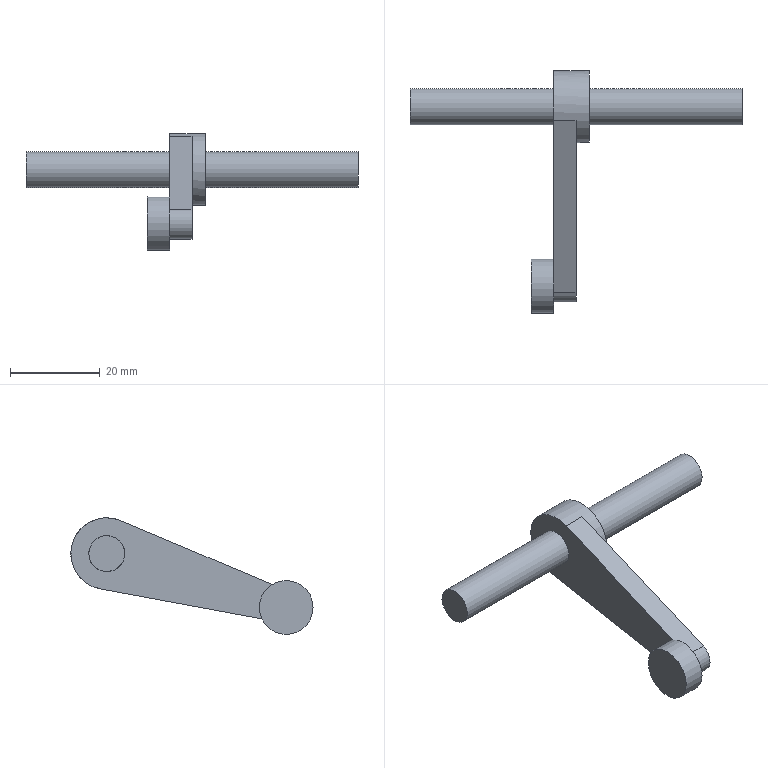Component | NX | DRIVEN_ROLLER | 3 solids | 17 faces | box 74 x 54 x 26 mm | volume 7500 mm3 | plane 10 | cylinder 7 | commonest cylinder face diameters 3 x2 8 x2 12 x1 7 x1 16 x1
STEP:
#1=CARTESIAN_POINT('',(0.,0.,0.));
#2=DIRECTION('',(0.,0.,1.));
#3=DIRECTION('',(1.,0.,0.));
#4=AXIS2_PLACEMENT_3D('',#1,#2,#3);
#5=CARTESIAN_POINT('',(25.,6.,197.818));
#6=VERTEX_POINT('',#5);
#7=CARTESIAN_POINT('',(25.,0.,197.818));
#8=DIRECTION('',(1.,0.,0.));
#9=DIRECTION('',(0.,1.,0.));
#10=AXIS2_PLACEMENT_3D('',#7,#8,#9);
#11=CIRCLE('',#10,6.);
#12=CARTESIAN_POINT('',(25.,0.,197.818));
#13=DIRECTION('',(-1.,0.,0.));
#14=DIRECTION('',(0.,0.,1.));
#15=AXIS2_PLACEMENT_3D('',#12,#13,#14);
#16=CYLINDRICAL_SURFACE('',#15,6.);
#17=CARTESIAN_POINT('',(7.854,0.));
#18=DIRECTION('',(-1.,0.));
#19=VECTOR('',#18,1.);
#20=LINE('',#17,#19);
#21=(GEOMETRIC_REPRESENTATION_CONTEXT(2)PARAMETRIC_REPRESENTATION_CONTEXT()REPRESENTATION_CONTEXT('',''));
#22=DEFINITIONAL_REPRESENTATION('',(#20),#21);
#23=PCURVE('',#16,#22);
#24=CARTESIAN_POINT('',(25.,0.,197.818));
#25=DIRECTION('',(1.,0.,0.));
#26=DIRECTION('',(0.,0.,-1.));
#27=AXIS2_PLACEMENT_3D('',#24,#25,#26);
#28=PLANE('',#27);
#29=CARTESIAN_POINT('',(0.,0.));
#30=DIRECTION('',(0.,1.));
#31=AXIS2_PLACEMENT_2D('',#29,#30);
#32=CIRCLE('',#31,6.);
#33=(GEOMETRIC_REPRESENTATION_CONTEXT(2)PARAMETRIC_REPRESENTATION_CONTEXT()REPRESENTATION_CONTEXT('',''));
#34=DEFINITIONAL_REPRESENTATION('',(#32),#33);
#35=PCURVE('',#28,#34);
#36=SURFACE_CURVE('',#11,(#23,#35),.PCURVE_S1.);
#37=EDGE_CURVE('',#6,#6,#36,.T.);
#38=ORIENTED_EDGE('',*,*,#37,.F.);
#39=CARTESIAN_POINT('',(20.,6.,197.818));
#40=VERTEX_POINT('',#39);
#41=CARTESIAN_POINT('',(25.,6.,197.818));
#42=CARTESIAN_POINT('',(20.,6.,197.818));
#43=B_SPLINE_CURVE_WITH_KNOTS('',1,(#41,#42),.UNSPECIFIED.,.F.,.F.,(2,2),(0.,5.),.PIECEWISE_BEZIER_KNOTS.);
#44=CARTESIAN_POINT('',(7.854,0.));
#45=DIRECTION('',(0.,1.));
#46=VECTOR('',#45,1.);
#47=LINE('',#44,#46);
#48=(GEOMETRIC_REPRESENTATION_CONTEXT(2)PARAMETRIC_REPRESENTATION_CONTEXT()REPRESENTATION_CONTEXT('',''));
#49=DEFINITIONAL_REPRESENTATION('',(#47),#48);
#50=PCURVE('',#16,#49);
#51=CARTESIAN_POINT('',(1.571,0.));
#52=DIRECTION('',(0.,1.));
#53=VECTOR('',#52,1.);
#54=LINE('',#51,#53);
#55=(GEOMETRIC_REPRESENTATION_CONTEXT(2)PARAMETRIC_REPRESENTATION_CONTEXT()REPRESENTATION_CONTEXT('',''));
#56=DEFINITIONAL_REPRESENTATION('',(#54),#55);
#57=PCURVE('',#16,#56);
#58=SEAM_CURVE('',#43,(#50,#57),.PCURVE_S1.);
#59=EDGE_CURVE('',#6,#40,#58,.T.);
#60=ORIENTED_EDGE('',*,*,#59,.T.);
#61=CARTESIAN_POINT('',(20.,0.,197.818));
#62=DIRECTION('',(1.,0.,0.));
#63=DIRECTION('',(0.,1.,0.));
#64=AXIS2_PLACEMENT_3D('',#61,#62,#63);
#65=CIRCLE('',#64,6.);
#66=CARTESIAN_POINT('',(7.854,5.));
#67=DIRECTION('',(-1.,0.));
#68=VECTOR('',#67,1.);
#69=LINE('',#66,#68);
#70=(GEOMETRIC_REPRESENTATION_CONTEXT(2)PARAMETRIC_REPRESENTATION_CONTEXT()REPRESENTATION_CONTEXT('',''));
#71=DEFINITIONAL_REPRESENTATION('',(#69),#70);
#72=PCURVE('',#16,#71);
#73=CARTESIAN_POINT('',(20.,0.,197.818));
#74=DIRECTION('',(1.,0.,0.));
#75=DIRECTION('',(0.,0.,-1.));
#76=AXIS2_PLACEMENT_3D('',#73,#74,#75);
#77=PLANE('',#76);
#78=CARTESIAN_POINT('',(0.,0.));
#79=DIRECTION('',(0.,1.));
#80=AXIS2_PLACEMENT_2D('',#78,#79);
#81=CIRCLE('',#80,6.);
#82=(GEOMETRIC_REPRESENTATION_CONTEXT(2)PARAMETRIC_REPRESENTATION_CONTEXT()REPRESENTATION_CONTEXT('',''));
#83=DEFINITIONAL_REPRESENTATION('',(#81),#82);
#84=PCURVE('',#77,#83);
#85=SURFACE_CURVE('',#65,(#72,#84),.PCURVE_S1.);
#86=EDGE_CURVE('',#40,#40,#85,.T.);
#87=ORIENTED_EDGE('',*,*,#86,.T.);
#88=ORIENTED_EDGE('',*,*,#59,.F.);
#89=EDGE_LOOP('',(#38,#60,#87,#88));
#90=FACE_BOUND('',#89,.T.);
#91=ADVANCED_FACE('',(#90),#16,.T.);
#92=CARTESIAN_POINT('',(25.,1.5,197.818));
#93=VERTEX_POINT('',#92);
#94=CARTESIAN_POINT('',(25.,0.,197.818));
#95=DIRECTION('',(1.,0.,0.));
#96=DIRECTION('',(0.,1.,0.));
#97=AXIS2_PLACEMENT_3D('',#94,#95,#96);
#98=CIRCLE('',#97,1.5);
#99=CARTESIAN_POINT('',(0.,0.));
#100=DIRECTION('',(0.,1.));
#101=AXIS2_PLACEMENT_2D('',#99,#100);
#102=CIRCLE('',#101,1.5);
#103=(GEOMETRIC_REPRESENTATION_CONTEXT(2)PARAMETRIC_REPRESENTATION_CONTEXT()REPRESENTATION_CONTEXT('',''));
#104=DEFINITIONAL_REPRESENTATION('',(#102),#103);
#105=PCURVE('',#28,#104);
#106=CARTESIAN_POINT('',(30.,0.,197.818));
#107=DIRECTION('',(-1.,0.,0.));
#108=DIRECTION('',(0.,0.,1.));
#109=AXIS2_PLACEMENT_3D('',#106,#107,#108);
#110=CYLINDRICAL_SURFACE('',#109,1.5);
#111=CARTESIAN_POINT('',(7.854,5.));
#112=DIRECTION('',(-1.,0.));
#113=VECTOR('',#112,1.);
#114=LINE('',#111,#113);
#115=(GEOMETRIC_REPRESENTATION_CONTEXT(2)PARAMETRIC_REPRESENTATION_CONTEXT()REPRESENTATION_CONTEXT('',''));
#116=DEFINITIONAL_REPRESENTATION('',(#114),#115);
#117=PCURVE('',#110,#116);
#118=SURFACE_CURVE('',#98,(#105,#117),.PCURVE_S1.);
#119=EDGE_CURVE('',#93,#93,#118,.T.);
#120=ORIENTED_EDGE('',*,*,#119,.F.);
#121=EDGE_LOOP('',(#120));
#122=FACE_BOUND('',#121,.T.);
#123=ORIENTED_EDGE('',*,*,#37,.T.);
#124=EDGE_LOOP('',(#123));
#125=FACE_BOUND('',#124,.T.);
#126=ADVANCED_FACE('',(#122,#125),#28,.T.);
#127=ORIENTED_EDGE('',*,*,#86,.F.);
#128=EDGE_LOOP('',(#127));
#129=FACE_BOUND('',#128,.T.);
#130=ADVANCED_FACE('',(#129),#77,.F.);
#131=CARTESIAN_POINT('',(30.,1.5,197.818));
#132=VERTEX_POINT('',#131);
#133=CARTESIAN_POINT('',(30.,0.,197.818));
#134=DIRECTION('',(1.,0.,0.));
#135=DIRECTION('',(0.,1.,0.));
#136=AXIS2_PLACEMENT_3D('',#133,#134,#135);
#137=CIRCLE('',#136,1.5);
#138=CARTESIAN_POINT('',(7.854,0.));
#139=DIRECTION('',(-1.,0.));
#140=VECTOR('',#139,1.);
#141=LINE('',#138,#140);
#142=(GEOMETRIC_REPRESENTATION_CONTEXT(2)PARAMETRIC_REPRESENTATION_CONTEXT()REPRESENTATION_CONTEXT('',''));
#143=DEFINITIONAL_REPRESENTATION('',(#141),#142);
#144=PCURVE('',#110,#143);
#145=CARTESIAN_POINT('',(30.,0.,197.818));
#146=DIRECTION('',(1.,0.,0.));
#147=DIRECTION('',(0.,0.,-1.));
#148=AXIS2_PLACEMENT_3D('',#145,#146,#147);
#149=PLANE('',#148);
#150=CARTESIAN_POINT('',(0.,0.));
#151=DIRECTION('',(0.,1.));
#152=AXIS2_PLACEMENT_2D('',#150,#151);
#153=CIRCLE('',#152,1.5);
#154=(GEOMETRIC_REPRESENTATION_CONTEXT(2)PARAMETRIC_REPRESENTATION_CONTEXT()REPRESENTATION_CONTEXT('',''));
#155=DEFINITIONAL_REPRESENTATION('',(#153),#154);
#156=PCURVE('',#149,#155);
#157=SURFACE_CURVE('',#137,(#144,#156),.PCURVE_S1.);
#158=EDGE_CURVE('',#132,#132,#157,.T.);
#159=ORIENTED_EDGE('',*,*,#158,.F.);
#160=CARTESIAN_POINT('',(30.,1.5,197.818));
#161=CARTESIAN_POINT('',(25.,1.5,197.818));
#162=B_SPLINE_CURVE_WITH_KNOTS('',1,(#160,#161),.UNSPECIFIED.,.F.,.F.,(2,2),(0.,5.),.PIECEWISE_BEZIER_KNOTS.);
#163=CARTESIAN_POINT('',(7.854,0.));
#164=DIRECTION('',(0.,1.));
#165=VECTOR('',#164,1.);
#166=LINE('',#163,#165);
#167=(GEOMETRIC_REPRESENTATION_CONTEXT(2)PARAMETRIC_REPRESENTATION_CONTEXT()REPRESENTATION_CONTEXT('',''));
#168=DEFINITIONAL_REPRESENTATION('',(#166),#167);
#169=PCURVE('',#110,#168);
#170=CARTESIAN_POINT('',(1.571,0.));
#171=DIRECTION('',(0.,1.));
#172=VECTOR('',#171,1.);
#173=LINE('',#170,#172);
#174=(GEOMETRIC_REPRESENTATION_CONTEXT(2)PARAMETRIC_REPRESENTATION_CONTEXT()REPRESENTATION_CONTEXT('',''));
#175=DEFINITIONAL_REPRESENTATION('',(#173),#174);
#176=PCURVE('',#110,#175);
#177=SEAM_CURVE('',#162,(#169,#176),.PCURVE_S1.);
#178=EDGE_CURVE('',#132,#93,#177,.T.);
#179=ORIENTED_EDGE('',*,*,#178,.T.);
#180=ORIENTED_EDGE('',*,*,#119,.T.);
#181=ORIENTED_EDGE('',*,*,#178,.F.);
#182=EDGE_LOOP('',(#159,#179,#180,#181));
#183=FACE_BOUND('',#182,.T.);
#184=ADVANCED_FACE('',(#183),#110,.T.);
#185=ORIENTED_EDGE('',*,*,#158,.T.);
#186=EDGE_LOOP('',(#185));
#187=FACE_BOUND('',#186,.T.);
#188=ADVANCED_FACE('',(#187),#149,.T.);
#189=CLOSED_SHELL('',(#91,#126,#130,#184,#188));
#190=MANIFOLD_SOLID_BREP('',#189);
#191=(LENGTH_UNIT()NAMED_UNIT(*)SI_UNIT(.MILLI.,.METRE.));
#192=UNCERTAINTY_MEASURE_WITH_UNIT(LENGTH_MEASURE(0.00001),#191,'','');
#193=(NAMED_UNIT(*)PLANE_ANGLE_UNIT()SI_UNIT($,.RADIAN.));
#194=(NAMED_UNIT(*)SI_UNIT($,.STERADIAN.)SOLID_ANGLE_UNIT());
#195=(GEOMETRIC_REPRESENTATION_CONTEXT(3)GLOBAL_UNCERTAINTY_ASSIGNED_CONTEXT((#192))GLOBAL_UNIT_ASSIGNED_CONTEXT((#191,#193,#194))REPRESENTATION_CONTEXT('',''));
#196=ADVANCED_BREP_SHAPE_REPRESENTATION('',(#4,#190),#195);
#197=CARTESIAN_POINT('',(0.,0.,0.));
#198=DIRECTION('',(0.,0.,1.));
#199=DIRECTION('',(1.,0.,0.));
#200=AXIS2_PLACEMENT_3D('',#197,#198,#199);
#201=CARTESIAN_POINT('',(0.,0.,0.));
#202=DIRECTION('',(0.,0.,1.));
#203=DIRECTION('',(1.,0.,0.));
#204=AXIS2_PLACEMENT_3D('',#201,#202,#203);
#205=CARTESIAN_POINT('',(0.,0.,0.));
#206=DIRECTION('',(0.,0.,1.));
#207=DIRECTION('',(1.,0.,0.));
#208=AXIS2_PLACEMENT_3D('',#205,#206,#207);
#209=(LENGTH_UNIT()NAMED_UNIT(*)SI_UNIT(.MILLI.,.METRE.));
#210=UNCERTAINTY_MEASURE_WITH_UNIT(LENGTH_MEASURE(0.000005),#209,'','');
#211=(NAMED_UNIT(*)PLANE_ANGLE_UNIT()SI_UNIT($,.RADIAN.));
#212=(NAMED_UNIT(*)SI_UNIT($,.STERADIAN.)SOLID_ANGLE_UNIT());
#213=(GEOMETRIC_REPRESENTATION_CONTEXT(3)GLOBAL_UNCERTAINTY_ASSIGNED_CONTEXT((#210))GLOBAL_UNIT_ASSIGNED_CONTEXT((#209,#211,#212))REPRESENTATION_CONTEXT('',''));
#214=SHAPE_REPRESENTATION('',(#4,#200,#204,#208),#213);
#215=ITEM_DEFINED_TRANSFORMATION('','',#4,#200);
#216=(REPRESENTATION_RELATIONSHIP('','',#196,#214)REPRESENTATION_RELATIONSHIP_WITH_TRANSFORMATION(#215)SHAPE_REPRESENTATION_RELATIONSHIP());
#217=CARTESIAN_POINT('',(25.,-1.361,201.043));
#218=VERTEX_POINT('',#217);
#219=CARTESIAN_POINT('',(25.,0.6386,194.377));
#220=VERTEX_POINT('',#219);
#221=CARTESIAN_POINT('',(25.,0.,197.818));
#222=DIRECTION('',(1.,0.,0.));
#223=DIRECTION('',(0.,1.,0.));
#224=AXIS2_PLACEMENT_3D('',#221,#222,#223);
#225=CIRCLE('',#224,3.5);
#226=CARTESIAN_POINT('',(30.,0.,197.818));
#227=DIRECTION('',(-1.,0.,0.));
#228=DIRECTION('',(0.,0.,1.));
#229=AXIS2_PLACEMENT_3D('',#226,#227,#228);
#230=CYLINDRICAL_SURFACE('',#229,3.5);
#231=CARTESIAN_POINT('',(7.854,5.));
#232=DIRECTION('',(-1.,0.));
#233=VECTOR('',#232,1.);
#234=LINE('',#231,#233);
#235=(GEOMETRIC_REPRESENTATION_CONTEXT(2)PARAMETRIC_REPRESENTATION_CONTEXT()REPRESENTATION_CONTEXT('',''));
#236=DEFINITIONAL_REPRESENTATION('',(#234),#235);
#237=PCURVE('',#230,#236);
#238=CARTESIAN_POINT('',(25.,0.,197.818));
#239=DIRECTION('',(1.,0.,0.));
#240=DIRECTION('',(0.,0.,-1.));
#241=AXIS2_PLACEMENT_3D('',#238,#239,#240);
#242=PLANE('',#241);
#243=CARTESIAN_POINT('',(0.,0.));
#244=DIRECTION('',(0.,1.));
#245=AXIS2_PLACEMENT_2D('',#243,#244);
#246=CIRCLE('',#245,3.5);
#247=(GEOMETRIC_REPRESENTATION_CONTEXT(2)PARAMETRIC_REPRESENTATION_CONTEXT()REPRESENTATION_CONTEXT('',''));
#248=DEFINITIONAL_REPRESENTATION('',(#246),#247);
#249=PCURVE('',#242,#248);
#250=SURFACE_CURVE('',#225,(#237,#249),.PCURVE_S1.);
#251=EDGE_CURVE('',#218,#220,#250,.T.);
#252=ORIENTED_EDGE('',*,*,#251,.T.);
#253=CARTESIAN_POINT('',(30.,0.6386,194.377));
#254=VERTEX_POINT('',#253);
#255=CARTESIAN_POINT('',(30.,0.6386,194.377));
#256=DIRECTION('',(-1.,0.,0.));
#257=VECTOR('',#256,1.);
#258=LINE('',#255,#257);
#259=CARTESIAN_POINT('',(2.958,0.));
#260=DIRECTION('',(0.,1.));
#261=VECTOR('',#260,1.);
#262=LINE('',#259,#261);
#263=(GEOMETRIC_REPRESENTATION_CONTEXT(2)PARAMETRIC_REPRESENTATION_CONTEXT()REPRESENTATION_CONTEXT('',''));
#264=DEFINITIONAL_REPRESENTATION('',(#262),#263);
#265=PCURVE('',#230,#264);
#266=CARTESIAN_POINT('',(30.,0.6386,194.377));
#267=DIRECTION('',(0.,-0.1825,0.9832));
#268=DIRECTION('',(0.,-0.9832,-0.1825));
#269=AXIS2_PLACEMENT_3D('',#266,#267,#268);
#270=PLANE('',#269);
#271=CARTESIAN_POINT('',(0.,0.));
#272=DIRECTION('',(0.,-1.));
#273=VECTOR('',#272,1.);
#274=LINE('',#271,#273);
#275=(GEOMETRIC_REPRESENTATION_CONTEXT(2)PARAMETRIC_REPRESENTATION_CONTEXT()REPRESENTATION_CONTEXT('',''));
#276=DEFINITIONAL_REPRESENTATION('',(#274),#275);
#277=PCURVE('',#270,#276);
#278=SURFACE_CURVE('',#258,(#265,#277),.PCURVE_S1.);
#279=EDGE_CURVE('',#254,#220,#278,.T.);
#280=ORIENTED_EDGE('',*,*,#279,.F.);
#281=CARTESIAN_POINT('',(30.,-1.361,201.043));
#282=VERTEX_POINT('',#281);
#283=CARTESIAN_POINT('',(30.,0.,197.818));
#284=DIRECTION('',(1.,0.,0.));
#285=DIRECTION('',(0.,1.,0.));
#286=AXIS2_PLACEMENT_3D('',#283,#284,#285);
#287=CIRCLE('',#286,3.5);
#288=CARTESIAN_POINT('',(7.854,0.));
#289=DIRECTION('',(-1.,0.));
#290=VECTOR('',#289,1.);
#291=LINE('',#288,#290);
#292=(GEOMETRIC_REPRESENTATION_CONTEXT(2)PARAMETRIC_REPRESENTATION_CONTEXT()REPRESENTATION_CONTEXT('',''));
#293=DEFINITIONAL_REPRESENTATION('',(#291),#292);
#294=PCURVE('',#230,#293);
#295=CARTESIAN_POINT('',(30.,0.,197.818));
#296=DIRECTION('',(1.,0.,0.));
#297=DIRECTION('',(0.,0.,-1.));
#298=AXIS2_PLACEMENT_3D('',#295,#296,#297);
#299=PLANE('',#298);
#300=CARTESIAN_POINT('',(0.,0.));
#301=DIRECTION('',(0.,1.));
#302=AXIS2_PLACEMENT_2D('',#300,#301);
#303=CIRCLE('',#302,3.5);
#304=(GEOMETRIC_REPRESENTATION_CONTEXT(2)PARAMETRIC_REPRESENTATION_CONTEXT()REPRESENTATION_CONTEXT('',''));
#305=DEFINITIONAL_REPRESENTATION('',(#303),#304);
#306=PCURVE('',#299,#305);
#307=SURFACE_CURVE('',#287,(#294,#306),.PCURVE_S1.);
#308=EDGE_CURVE('',#282,#254,#307,.T.);
#309=ORIENTED_EDGE('',*,*,#308,.F.);
#310=CARTESIAN_POINT('',(30.,-1.361,201.043));
#311=DIRECTION('',(-1.,0.,0.));
#312=VECTOR('',#311,1.);
#313=LINE('',#310,#312);
#314=CARTESIAN_POINT('',(5.884,0.));
#315=DIRECTION('',(0.,1.));
#316=VECTOR('',#315,1.);
#317=LINE('',#314,#316);
#318=(GEOMETRIC_REPRESENTATION_CONTEXT(2)PARAMETRIC_REPRESENTATION_CONTEXT()REPRESENTATION_CONTEXT('',''));
#319=DEFINITIONAL_REPRESENTATION('',(#317),#318);
#320=PCURVE('',#230,#319);
#321=CARTESIAN_POINT('',(30.,36.889,217.189));
#322=DIRECTION('',(0.,0.3889,-0.9213));
#323=DIRECTION('',(0.,0.9213,0.3889));
#324=AXIS2_PLACEMENT_3D('',#321,#322,#323);
#325=PLANE('',#324);
#326=CARTESIAN_POINT('',(-41.518,0.));
#327=DIRECTION('',(0.,-1.));
#328=VECTOR('',#327,1.);
#329=LINE('',#326,#328);
#330=(GEOMETRIC_REPRESENTATION_CONTEXT(2)PARAMETRIC_REPRESENTATION_CONTEXT()REPRESENTATION_CONTEXT('',''));
#331=DEFINITIONAL_REPRESENTATION('',(#329),#330);
#332=PCURVE('',#325,#331);
#333=SURFACE_CURVE('',#313,(#320,#332),.PCURVE_S1.);
#334=EDGE_CURVE('',#282,#218,#333,.T.);
#335=ORIENTED_EDGE('',*,*,#334,.T.);
#336=EDGE_LOOP('',(#252,#280,#309,#335));
#337=FACE_BOUND('',#336,.T.);
#338=ADVANCED_FACE('',(#337),#230,.T.);
#339=CARTESIAN_POINT('',(25.,41.46,201.953));
#340=VERTEX_POINT('',#339);
#341=CARTESIAN_POINT('',(25.,0.6386,194.377));
#342=DIRECTION('',(0.,0.9832,0.1825));
#343=VECTOR('',#342,1.);
#344=LINE('',#341,#343);
#345=CARTESIAN_POINT('',(0.,-5.));
#346=DIRECTION('',(-1.,0.));
#347=VECTOR('',#346,1.);
#348=LINE('',#345,#347);
#349=(GEOMETRIC_REPRESENTATION_CONTEXT(2)PARAMETRIC_REPRESENTATION_CONTEXT()REPRESENTATION_CONTEXT('',''));
#350=DEFINITIONAL_REPRESENTATION('',(#348),#349);
#351=PCURVE('',#270,#350);
#352=CARTESIAN_POINT('',(3.441,0.6386));
#353=DIRECTION('',(-0.1825,0.9832));
#354=VECTOR('',#353,1.);
#355=LINE('',#352,#354);
#356=(GEOMETRIC_REPRESENTATION_CONTEXT(2)PARAMETRIC_REPRESENTATION_CONTEXT()REPRESENTATION_CONTEXT('',''));
#357=DEFINITIONAL_REPRESENTATION('',(#355),#356);
#358=PCURVE('',#242,#357);
#359=SURFACE_CURVE('',#344,(#351,#358),.PCURVE_S1.);
#360=EDGE_CURVE('',#220,#340,#359,.T.);
#361=ORIENTED_EDGE('',*,*,#360,.T.);
#362=CARTESIAN_POINT('',(30.,41.46,201.953));
#363=VERTEX_POINT('',#362);
#364=CARTESIAN_POINT('',(30.,41.46,201.953));
#365=DIRECTION('',(-1.,0.,0.));
#366=VECTOR('',#365,1.);
#367=LINE('',#364,#366);
#368=CARTESIAN_POINT('',(-41.518,0.));
#369=DIRECTION('',(0.,-1.));
#370=VECTOR('',#369,1.);
#371=LINE('',#368,#370);
#372=(GEOMETRIC_REPRESENTATION_CONTEXT(2)PARAMETRIC_REPRESENTATION_CONTEXT()REPRESENTATION_CONTEXT('',''));
#373=DEFINITIONAL_REPRESENTATION('',(#371),#372);
#374=PCURVE('',#270,#373);
#375=CARTESIAN_POINT('',(30.,40.,209.818));
#376=DIRECTION('',(-1.,0.,0.));
#377=DIRECTION('',(0.,0.,1.));
#378=AXIS2_PLACEMENT_3D('',#375,#376,#377);
#379=CYLINDRICAL_SURFACE('',#378,8.);
#380=CARTESIAN_POINT('',(9.241,0.));
#381=DIRECTION('',(0.,1.));
#382=VECTOR('',#381,1.);
#383=LINE('',#380,#382);
#384=(GEOMETRIC_REPRESENTATION_CONTEXT(2)PARAMETRIC_REPRESENTATION_CONTEXT()REPRESENTATION_CONTEXT('',''));
#385=DEFINITIONAL_REPRESENTATION('',(#383),#384);
#386=PCURVE('',#379,#385);
#387=SURFACE_CURVE('',#367,(#374,#386),.PCURVE_S1.);
#388=EDGE_CURVE('',#363,#340,#387,.T.);
#389=ORIENTED_EDGE('',*,*,#388,.F.);
#390=CARTESIAN_POINT('',(30.,0.6386,194.377));
#391=DIRECTION('',(0.,0.9832,0.1825));
#392=VECTOR('',#391,1.);
#393=LINE('',#390,#392);
#394=CARTESIAN_POINT('',(0.,0.));
#395=DIRECTION('',(-1.,0.));
#396=VECTOR('',#395,1.);
#397=LINE('',#394,#396);
#398=(GEOMETRIC_REPRESENTATION_CONTEXT(2)PARAMETRIC_REPRESENTATION_CONTEXT()REPRESENTATION_CONTEXT('',''));
#399=DEFINITIONAL_REPRESENTATION('',(#397),#398);
#400=PCURVE('',#270,#399);
#401=CARTESIAN_POINT('',(3.441,0.6386));
#402=DIRECTION('',(-0.1825,0.9832));
#403=VECTOR('',#402,1.);
#404=LINE('',#401,#403);
#405=(GEOMETRIC_REPRESENTATION_CONTEXT(2)PARAMETRIC_REPRESENTATION_CONTEXT()REPRESENTATION_CONTEXT('',''));
#406=DEFINITIONAL_REPRESENTATION('',(#404),#405);
#407=PCURVE('',#299,#406);
#408=SURFACE_CURVE('',#393,(#400,#407),.PCURVE_S1.);
#409=EDGE_CURVE('',#254,#363,#408,.T.);
#410=ORIENTED_EDGE('',*,*,#409,.F.);
#411=ORIENTED_EDGE('',*,*,#279,.T.);
#412=EDGE_LOOP('',(#361,#389,#410,#411));
#413=FACE_BOUND('',#412,.T.);
#414=ADVANCED_FACE('',(#413),#270,.F.);
#415=CARTESIAN_POINT('',(25.,36.889,217.189));
#416=VERTEX_POINT('',#415);
#417=CARTESIAN_POINT('',(25.,40.,209.818));
#418=DIRECTION('',(1.,0.,0.));
#419=DIRECTION('',(0.,1.,0.));
#420=AXIS2_PLACEMENT_3D('',#417,#418,#419);
#421=CIRCLE('',#420,8.);
#422=CARTESIAN_POINT('',(14.137,5.));
#423=DIRECTION('',(-1.,0.));
#424=VECTOR('',#423,1.);
#425=LINE('',#422,#424);
#426=(GEOMETRIC_REPRESENTATION_CONTEXT(2)PARAMETRIC_REPRESENTATION_CONTEXT()REPRESENTATION_CONTEXT('',''));
#427=DEFINITIONAL_REPRESENTATION('',(#425),#426);
#428=PCURVE('',#379,#427);
#429=CARTESIAN_POINT('',(-12.,40.));
#430=DIRECTION('',(0.,1.));
#431=AXIS2_PLACEMENT_2D('',#429,#430);
#432=CIRCLE('',#431,8.);
#433=(GEOMETRIC_REPRESENTATION_CONTEXT(2)PARAMETRIC_REPRESENTATION_CONTEXT()REPRESENTATION_CONTEXT('',''));
#434=DEFINITIONAL_REPRESENTATION('',(#432),#433);
#435=PCURVE('',#242,#434);
#436=SURFACE_CURVE('',#421,(#428,#435),.PCURVE_S1.);
#437=EDGE_CURVE('',#340,#416,#436,.T.);
#438=ORIENTED_EDGE('',*,*,#437,.T.);
#439=CARTESIAN_POINT('',(30.,36.889,217.189));
#440=VERTEX_POINT('',#439);
#441=CARTESIAN_POINT('',(30.,36.889,217.189));
#442=DIRECTION('',(-1.,0.,0.));
#443=VECTOR('',#442,1.);
#444=LINE('',#441,#443);
#445=CARTESIAN_POINT('',(5.884,0.));
#446=DIRECTION('',(0.,1.));
#447=VECTOR('',#446,1.);
#448=LINE('',#445,#447);
#449=(GEOMETRIC_REPRESENTATION_CONTEXT(2)PARAMETRIC_REPRESENTATION_CONTEXT()REPRESENTATION_CONTEXT('',''));
#450=DEFINITIONAL_REPRESENTATION('',(#448),#449);
#451=PCURVE('',#379,#450);
#452=CARTESIAN_POINT('',(-0.,0.));
#453=DIRECTION('',(0.,-1.));
#454=VECTOR('',#453,1.);
#455=LINE('',#452,#454);
#456=(GEOMETRIC_REPRESENTATION_CONTEXT(2)PARAMETRIC_REPRESENTATION_CONTEXT()REPRESENTATION_CONTEXT('',''));
#457=DEFINITIONAL_REPRESENTATION('',(#455),#456);
#458=PCURVE('',#325,#457);
#459=SURFACE_CURVE('',#444,(#451,#458),.PCURVE_S1.);
#460=EDGE_CURVE('',#440,#416,#459,.T.);
#461=ORIENTED_EDGE('',*,*,#460,.F.);
#462=CARTESIAN_POINT('',(33.,36.889,217.189));
#463=VERTEX_POINT('',#462);
#464=CARTESIAN_POINT('',(33.,36.889,217.189));
#465=CARTESIAN_POINT('',(30.,36.889,217.189));
#466=B_SPLINE_CURVE_WITH_KNOTS('',1,(#464,#465),.UNSPECIFIED.,.F.,.F.,(2,2),(-3.,0.),.PIECEWISE_BEZIER_KNOTS.);
#467=CARTESIAN_POINT('',(5.884,0.));
#468=DIRECTION('',(0.,1.));
#469=VECTOR('',#468,1.);
#470=LINE('',#467,#469);
#471=(GEOMETRIC_REPRESENTATION_CONTEXT(2)PARAMETRIC_REPRESENTATION_CONTEXT()REPRESENTATION_CONTEXT('',''));
#472=DEFINITIONAL_REPRESENTATION('',(#470),#471);
#473=PCURVE('',#379,#472);
#474=CARTESIAN_POINT('',(12.167,0.));
#475=DIRECTION('',(0.,1.));
#476=VECTOR('',#475,1.);
#477=LINE('',#474,#476);
#478=(GEOMETRIC_REPRESENTATION_CONTEXT(2)PARAMETRIC_REPRESENTATION_CONTEXT()REPRESENTATION_CONTEXT('',''));
#479=DEFINITIONAL_REPRESENTATION('',(#477),#478);
#480=PCURVE('',#379,#479);
#481=SEAM_CURVE('',#466,(#473,#480),.PCURVE_S1.);
#482=EDGE_CURVE('',#463,#440,#481,.T.);
#483=ORIENTED_EDGE('',*,*,#482,.F.);
#484=CARTESIAN_POINT('',(33.,47.866,211.278));
#485=VERTEX_POINT('',#484);
#486=CARTESIAN_POINT('',(33.,40.,209.818));
#487=DIRECTION('',(1.,0.,0.));
#488=DIRECTION('',(0.,0.9832,0.1825));
#489=AXIS2_PLACEMENT_3D('',#486,#487,#488);
#490=CIRCLE('',#489,8.);
#491=CARTESIAN_POINT('',(7.67,-3.));
#492=DIRECTION('',(-1.,0.));
#493=VECTOR('',#492,1.);
#494=LINE('',#491,#493);
#495=(GEOMETRIC_REPRESENTATION_CONTEXT(2)PARAMETRIC_REPRESENTATION_CONTEXT()REPRESENTATION_CONTEXT('',''));
#496=DEFINITIONAL_REPRESENTATION('',(#494),#495);
#497=PCURVE('',#379,#496);
#498=CARTESIAN_POINT('',(33.,40.,209.818));
#499=DIRECTION('',(1.,0.,0.));
#500=DIRECTION('',(0.,0.,-1.));
#501=AXIS2_PLACEMENT_3D('',#498,#499,#500);
#502=PLANE('',#501);
#503=CARTESIAN_POINT('',(0.,0.));
#504=DIRECTION('',(-0.1825,0.9832));
#505=AXIS2_PLACEMENT_2D('',#503,#504);
#506=CIRCLE('',#505,8.);
#507=(GEOMETRIC_REPRESENTATION_CONTEXT(2)PARAMETRIC_REPRESENTATION_CONTEXT()REPRESENTATION_CONTEXT('',''));
#508=DEFINITIONAL_REPRESENTATION('',(#506),#507);
#509=PCURVE('',#502,#508);
#510=SURFACE_CURVE('',#490,(#497,#509),.PCURVE_S1.);
#511=EDGE_CURVE('',#485,#463,#510,.T.);
#512=ORIENTED_EDGE('',*,*,#511,.F.);
#513=CARTESIAN_POINT('',(33.,40.,209.818));
#514=DIRECTION('',(1.,0.,0.));
#515=DIRECTION('',(0.,0.9832,0.1825));
#516=AXIS2_PLACEMENT_3D('',#513,#514,#515);
#517=CIRCLE('',#516,8.);
#518=CARTESIAN_POINT('',(13.954,-3.));
#519=DIRECTION('',(-1.,0.));
#520=VECTOR('',#519,1.);
#521=LINE('',#518,#520);
#522=(GEOMETRIC_REPRESENTATION_CONTEXT(2)PARAMETRIC_REPRESENTATION_CONTEXT()REPRESENTATION_CONTEXT('',''));
#523=DEFINITIONAL_REPRESENTATION('',(#521),#522);
#524=PCURVE('',#379,#523);
#525=CARTESIAN_POINT('',(0.,0.));
#526=DIRECTION('',(-0.1825,0.9832));
#527=AXIS2_PLACEMENT_2D('',#525,#526);
#528=CIRCLE('',#527,8.);
#529=(GEOMETRIC_REPRESENTATION_CONTEXT(2)PARAMETRIC_REPRESENTATION_CONTEXT()REPRESENTATION_CONTEXT('',''));
#530=DEFINITIONAL_REPRESENTATION('',(#528),#529);
#531=PCURVE('',#502,#530);
#532=SURFACE_CURVE('',#517,(#524,#531),.PCURVE_S1.);
#533=EDGE_CURVE('',#463,#485,#532,.T.);
#534=ORIENTED_EDGE('',*,*,#533,.F.);
#535=ORIENTED_EDGE('',*,*,#482,.T.);
#536=CARTESIAN_POINT('',(30.,40.,209.818));
#537=DIRECTION('',(-1.,0.,0.));
#538=DIRECTION('',(0.,0.9832,0.1825));
#539=AXIS2_PLACEMENT_3D('',#536,#537,#538);
#540=CIRCLE('',#539,8.);
#541=CARTESIAN_POINT('',(7.67,0.));
#542=DIRECTION('',(1.,0.));
#543=VECTOR('',#542,1.);
#544=LINE('',#541,#543);
#545=(GEOMETRIC_REPRESENTATION_CONTEXT(2)PARAMETRIC_REPRESENTATION_CONTEXT()REPRESENTATION_CONTEXT('',''));
#546=DEFINITIONAL_REPRESENTATION('',(#544),#545);
#547=PCURVE('',#379,#546);
#548=CARTESIAN_POINT('',(-13.46,47.866));
#549=CARTESIAN_POINT('',(0.1641,50.394));
#550=CARTESIAN_POINT('',(-4.458,37.331));
#551=CARTESIAN_POINT('',(-9.081,24.269));
#552=CARTESIAN_POINT('',(-18.082,34.803));
#553=CARTESIAN_POINT('',(-27.084,45.337));
#554=CARTESIAN_POINT('',(-13.46,47.866));
#555=(BOUNDED_CURVE()B_SPLINE_CURVE(2,(#548,#549,#550,#551,#552,#553,#554),.UNSPECIFIED.,.T.,.F.)B_SPLINE_CURVE_WITH_KNOTS((1,2,2,2,2,1),(-2.094,0.,2.094,4.189,6.283,8.378),.UNSPECIFIED.)CURVE()GEOMETRIC_REPRESENTATION_ITEM()RATIONAL_B_SPLINE_CURVE((1.,0.5,1.,0.5,1.,0.5,1.))REPRESENTATION_ITEM(''));
#556=(GEOMETRIC_REPRESENTATION_CONTEXT(2)PARAMETRIC_REPRESENTATION_CONTEXT()REPRESENTATION_CONTEXT('',''));
#557=DEFINITIONAL_REPRESENTATION('',(#555),#556);
#558=PCURVE('',#299,#557);
#559=SURFACE_CURVE('',#540,(#547,#558),.PCURVE_S1.);
#560=EDGE_CURVE('',#363,#440,#559,.T.);
#561=ORIENTED_EDGE('',*,*,#560,.F.);
#562=ORIENTED_EDGE('',*,*,#388,.T.);
#563=EDGE_LOOP('',(#438,#461,#483,#512,#534,#535,#561,#562));
#564=FACE_BOUND('',#563,.T.);
#565=ADVANCED_FACE('',(#564),#379,.T.);
#566=CARTESIAN_POINT('',(30.,1.5,197.818));
#567=VERTEX_POINT('',#566);
#568=CARTESIAN_POINT('',(30.,0.,197.818));
#569=DIRECTION('',(1.,0.,0.));
#570=DIRECTION('',(0.,1.,0.));
#571=AXIS2_PLACEMENT_3D('',#568,#569,#570);
#572=CIRCLE('',#571,1.5);
#573=CARTESIAN_POINT('',(30.,0.,197.818));
#574=DIRECTION('',(-1.,0.,0.));
#575=DIRECTION('',(0.,0.,1.));
#576=AXIS2_PLACEMENT_3D('',#573,#574,#575);
#577=CYLINDRICAL_SURFACE('',#576,1.5);
#578=CARTESIAN_POINT('',(7.854,0.));
#579=DIRECTION('',(-1.,0.));
#580=VECTOR('',#579,1.);
#581=LINE('',#578,#580);
#582=(GEOMETRIC_REPRESENTATION_CONTEXT(2)PARAMETRIC_REPRESENTATION_CONTEXT()REPRESENTATION_CONTEXT('',''));
#583=DEFINITIONAL_REPRESENTATION('',(#581),#582);
#584=PCURVE('',#577,#583);
#585=CARTESIAN_POINT('',(0.,0.));
#586=DIRECTION('',(0.,1.));
#587=AXIS2_PLACEMENT_2D('',#585,#586);
#588=CIRCLE('',#587,1.5);
#589=(GEOMETRIC_REPRESENTATION_CONTEXT(2)PARAMETRIC_REPRESENTATION_CONTEXT()REPRESENTATION_CONTEXT('',''));
#590=DEFINITIONAL_REPRESENTATION('',(#588),#589);
#591=PCURVE('',#299,#590);
#592=SURFACE_CURVE('',#572,(#584,#591),.PCURVE_S1.);
#593=EDGE_CURVE('',#567,#567,#592,.T.);
#594=ORIENTED_EDGE('',*,*,#593,.F.);
#595=CARTESIAN_POINT('',(25.,1.5,197.818));
#596=VERTEX_POINT('',#595);
#597=CARTESIAN_POINT('',(30.,1.5,197.818));
#598=CARTESIAN_POINT('',(25.,1.5,197.818));
#599=B_SPLINE_CURVE_WITH_KNOTS('',1,(#597,#598),.UNSPECIFIED.,.F.,.F.,(2,2),(0.,5.),.PIECEWISE_BEZIER_KNOTS.);
#600=CARTESIAN_POINT('',(7.854,0.));
#601=DIRECTION('',(0.,1.));
#602=VECTOR('',#601,1.);
#603=LINE('',#600,#602);
#604=(GEOMETRIC_REPRESENTATION_CONTEXT(2)PARAMETRIC_REPRESENTATION_CONTEXT()REPRESENTATION_CONTEXT('',''));
#605=DEFINITIONAL_REPRESENTATION('',(#603),#604);
#606=PCURVE('',#577,#605);
#607=CARTESIAN_POINT('',(1.571,0.));
#608=DIRECTION('',(0.,1.));
#609=VECTOR('',#608,1.);
#610=LINE('',#607,#609);
#611=(GEOMETRIC_REPRESENTATION_CONTEXT(2)PARAMETRIC_REPRESENTATION_CONTEXT()REPRESENTATION_CONTEXT('',''));
#612=DEFINITIONAL_REPRESENTATION('',(#610),#611);
#613=PCURVE('',#577,#612);
#614=SEAM_CURVE('',#599,(#606,#613),.PCURVE_S1.);
#615=EDGE_CURVE('',#567,#596,#614,.T.);
#616=ORIENTED_EDGE('',*,*,#615,.T.);
#617=CARTESIAN_POINT('',(25.,0.,197.818));
#618=DIRECTION('',(1.,0.,0.));
#619=DIRECTION('',(0.,1.,0.));
#620=AXIS2_PLACEMENT_3D('',#617,#618,#619);
#621=CIRCLE('',#620,1.5);
#622=CARTESIAN_POINT('',(7.854,5.));
#623=DIRECTION('',(-1.,0.));
#624=VECTOR('',#623,1.);
#625=LINE('',#622,#624);
#626=(GEOMETRIC_REPRESENTATION_CONTEXT(2)PARAMETRIC_REPRESENTATION_CONTEXT()REPRESENTATION_CONTEXT('',''));
#627=DEFINITIONAL_REPRESENTATION('',(#625),#626);
#628=PCURVE('',#577,#627);
#629=CARTESIAN_POINT('',(0.,0.));
#630=DIRECTION('',(0.,1.));
#631=AXIS2_PLACEMENT_2D('',#629,#630);
#632=CIRCLE('',#631,1.5);
#633=(GEOMETRIC_REPRESENTATION_CONTEXT(2)PARAMETRIC_REPRESENTATION_CONTEXT()REPRESENTATION_CONTEXT('',''));
#634=DEFINITIONAL_REPRESENTATION('',(#632),#633);
#635=PCURVE('',#242,#634);
#636=SURFACE_CURVE('',#621,(#628,#635),.PCURVE_S1.);
#637=EDGE_CURVE('',#596,#596,#636,.T.);
#638=ORIENTED_EDGE('',*,*,#637,.T.);
#639=ORIENTED_EDGE('',*,*,#615,.F.);
#640=EDGE_LOOP('',(#594,#616,#638,#639));
#641=FACE_BOUND('',#640,.F.);
#642=ADVANCED_FACE('',(#641),#577,.F.);
#643=CARTESIAN_POINT('',(25.,36.889,217.189));
#644=DIRECTION('',(0.,-0.9213,-0.3889));
#645=VECTOR('',#644,1.);
#646=LINE('',#643,#645);
#647=CARTESIAN_POINT('',(0.,-5.));
#648=DIRECTION('',(-1.,0.));
#649=VECTOR('',#648,1.);
#650=LINE('',#647,#649);
#651=(GEOMETRIC_REPRESENTATION_CONTEXT(2)PARAMETRIC_REPRESENTATION_CONTEXT()REPRESENTATION_CONTEXT('',''));
#652=DEFINITIONAL_REPRESENTATION('',(#650),#651);
#653=PCURVE('',#325,#652);
#654=CARTESIAN_POINT('',(-19.37,36.889));
#655=DIRECTION('',(0.3889,-0.9213));
#656=VECTOR('',#655,1.);
#657=LINE('',#654,#656);
#658=(GEOMETRIC_REPRESENTATION_CONTEXT(2)PARAMETRIC_REPRESENTATION_CONTEXT()REPRESENTATION_CONTEXT('',''));
#659=DEFINITIONAL_REPRESENTATION('',(#657),#658);
#660=PCURVE('',#242,#659);
#661=SURFACE_CURVE('',#646,(#653,#660),.PCURVE_S1.);
#662=EDGE_CURVE('',#416,#218,#661,.T.);
#663=ORIENTED_EDGE('',*,*,#662,.T.);
#664=ORIENTED_EDGE('',*,*,#334,.F.);
#665=CARTESIAN_POINT('',(30.,36.889,217.189));
#666=DIRECTION('',(0.,-0.9213,-0.3889));
#667=VECTOR('',#666,1.);
#668=LINE('',#665,#667);
#669=CARTESIAN_POINT('',(0.,0.));
#670=DIRECTION('',(-1.,0.));
#671=VECTOR('',#670,1.);
#672=LINE('',#669,#671);
#673=(GEOMETRIC_REPRESENTATION_CONTEXT(2)PARAMETRIC_REPRESENTATION_CONTEXT()REPRESENTATION_CONTEXT('',''));
#674=DEFINITIONAL_REPRESENTATION('',(#672),#673);
#675=PCURVE('',#325,#674);
#676=CARTESIAN_POINT('',(-19.37,36.889));
#677=DIRECTION('',(0.3889,-0.9213));
#678=VECTOR('',#677,1.);
#679=LINE('',#676,#678);
#680=(GEOMETRIC_REPRESENTATION_CONTEXT(2)PARAMETRIC_REPRESENTATION_CONTEXT()REPRESENTATION_CONTEXT('',''));
#681=DEFINITIONAL_REPRESENTATION('',(#679),#680);
#682=PCURVE('',#299,#681);
#683=SURFACE_CURVE('',#668,(#675,#682),.PCURVE_S1.);
#684=EDGE_CURVE('',#440,#282,#683,.T.);
#685=ORIENTED_EDGE('',*,*,#684,.F.);
#686=ORIENTED_EDGE('',*,*,#460,.T.);
#687=EDGE_LOOP('',(#663,#664,#685,#686));
#688=FACE_BOUND('',#687,.T.);
#689=ADVANCED_FACE('',(#688),#325,.F.);
#690=CARTESIAN_POINT('',(25.,44.,209.818));
#691=VERTEX_POINT('',#690);
#692=CARTESIAN_POINT('',(25.,43.933,210.548));
#693=VERTEX_POINT('',#692);
#694=CARTESIAN_POINT('',(25.,40.,209.818));
#695=DIRECTION('',(1.,0.,0.));
#696=DIRECTION('',(0.,1.,0.));
#697=AXIS2_PLACEMENT_3D('',#694,#695,#696);
#698=CIRCLE('',#697,4.);
#699=CARTESIAN_POINT('',(30.,40.,209.818));
#700=DIRECTION('',(-1.,0.,0.));
#701=DIRECTION('',(0.,0.,1.));
#702=AXIS2_PLACEMENT_3D('',#699,#700,#701);
#703=CYLINDRICAL_SURFACE('',#702,4.);
#704=CARTESIAN_POINT('',(1.571,5.));
#705=DIRECTION('',(-1.,0.));
#706=VECTOR('',#705,1.);
#707=LINE('',#704,#706);
#708=(GEOMETRIC_REPRESENTATION_CONTEXT(2)PARAMETRIC_REPRESENTATION_CONTEXT()REPRESENTATION_CONTEXT('',''));
#709=DEFINITIONAL_REPRESENTATION('',(#707),#708);
#710=PCURVE('',#703,#709);
#711=CARTESIAN_POINT('',(-12.,40.));
#712=DIRECTION('',(0.,1.));
#713=AXIS2_PLACEMENT_2D('',#711,#712);
#714=CIRCLE('',#713,4.);
#715=(GEOMETRIC_REPRESENTATION_CONTEXT(2)PARAMETRIC_REPRESENTATION_CONTEXT()REPRESENTATION_CONTEXT('',''));
#716=DEFINITIONAL_REPRESENTATION('',(#714),#715);
#717=PCURVE('',#242,#716);
#718=SURFACE_CURVE('',#698,(#710,#717),.PCURVE_S1.);
#719=EDGE_CURVE('',#691,#693,#718,.T.);
#720=ORIENTED_EDGE('',*,*,#719,.T.);
#721=CARTESIAN_POINT('',(33.,43.933,210.548));
#722=VERTEX_POINT('',#721);
#723=CARTESIAN_POINT('',(33.,43.933,210.548));
#724=CARTESIAN_POINT('',(25.,43.933,210.548));
#725=B_SPLINE_CURVE_WITH_KNOTS('',1,(#723,#724),.UNSPECIFIED.,.F.,.F.,(2,2),(-3.,5.),.PIECEWISE_BEZIER_KNOTS.);
#726=CARTESIAN_POINT('',(1.387,0.));
#727=DIRECTION('',(0.,1.));
#728=VECTOR('',#727,1.);
#729=LINE('',#726,#728);
#730=(GEOMETRIC_REPRESENTATION_CONTEXT(2)PARAMETRIC_REPRESENTATION_CONTEXT()REPRESENTATION_CONTEXT('',''));
#731=DEFINITIONAL_REPRESENTATION('',(#729),#730);
#732=PCURVE('',#703,#731);
#733=CARTESIAN_POINT('',(7.67,0.));
#734=DIRECTION('',(0.,1.));
#735=VECTOR('',#734,1.);
#736=LINE('',#733,#735);
#737=(GEOMETRIC_REPRESENTATION_CONTEXT(2)PARAMETRIC_REPRESENTATION_CONTEXT()REPRESENTATION_CONTEXT('',''));
#738=DEFINITIONAL_REPRESENTATION('',(#736),#737);
#739=PCURVE('',#703,#738);
#740=SEAM_CURVE('',#725,(#732,#739),.PCURVE_S1.);
#741=EDGE_CURVE('',#722,#693,#740,.T.);
#742=ORIENTED_EDGE('',*,*,#741,.F.);
#743=CARTESIAN_POINT('',(33.,40.,209.818));
#744=DIRECTION('',(1.,0.,0.));
#745=DIRECTION('',(0.,0.9832,0.1825));
#746=AXIS2_PLACEMENT_3D('',#743,#744,#745);
#747=CIRCLE('',#746,4.);
#748=CARTESIAN_POINT('',(7.67,-3.));
#749=DIRECTION('',(-1.,0.));
#750=VECTOR('',#749,1.);
#751=LINE('',#748,#750);
#752=(GEOMETRIC_REPRESENTATION_CONTEXT(2)PARAMETRIC_REPRESENTATION_CONTEXT()REPRESENTATION_CONTEXT('',''));
#753=DEFINITIONAL_REPRESENTATION('',(#751),#752);
#754=PCURVE('',#703,#753);
#755=CARTESIAN_POINT('',(0.,0.));
#756=DIRECTION('',(-0.1825,0.9832));
#757=AXIS2_PLACEMENT_2D('',#755,#756);
#758=CIRCLE('',#757,4.);
#759=(GEOMETRIC_REPRESENTATION_CONTEXT(2)PARAMETRIC_REPRESENTATION_CONTEXT()REPRESENTATION_CONTEXT('',''));
#760=DEFINITIONAL_REPRESENTATION('',(#758),#759);
#761=PCURVE('',#502,#760);
#762=SURFACE_CURVE('',#747,(#754,#761),.PCURVE_S1.);
#763=EDGE_CURVE('',#722,#722,#762,.T.);
#764=ORIENTED_EDGE('',*,*,#763,.F.);
#765=ORIENTED_EDGE('',*,*,#741,.T.);
#766=CARTESIAN_POINT('',(25.,40.,209.818));
#767=DIRECTION('',(1.,0.,0.));
#768=DIRECTION('',(0.,1.,0.));
#769=AXIS2_PLACEMENT_3D('',#766,#767,#768);
#770=CIRCLE('',#769,4.);
#771=CARTESIAN_POINT('',(7.854,5.));
#772=DIRECTION('',(-1.,0.));
#773=VECTOR('',#772,1.);
#774=LINE('',#771,#773);
#775=(GEOMETRIC_REPRESENTATION_CONTEXT(2)PARAMETRIC_REPRESENTATION_CONTEXT()REPRESENTATION_CONTEXT('',''));
#776=DEFINITIONAL_REPRESENTATION('',(#774),#775);
#777=PCURVE('',#703,#776);
#778=CARTESIAN_POINT('',(-12.,40.));
#779=DIRECTION('',(0.,1.));
#780=AXIS2_PLACEMENT_2D('',#778,#779);
#781=CIRCLE('',#780,4.);
#782=(GEOMETRIC_REPRESENTATION_CONTEXT(2)PARAMETRIC_REPRESENTATION_CONTEXT()REPRESENTATION_CONTEXT('',''));
#783=DEFINITIONAL_REPRESENTATION('',(#781),#782);
#784=PCURVE('',#242,#783);
#785=SURFACE_CURVE('',#770,(#777,#784),.PCURVE_S1.);
#786=EDGE_CURVE('',#693,#691,#785,.T.);
#787=ORIENTED_EDGE('',*,*,#786,.T.);
#788=EDGE_LOOP('',(#720,#742,#764,#765,#787));
#789=FACE_BOUND('',#788,.F.);
#790=ADVANCED_FACE('',(#789),#703,.F.);
#791=ORIENTED_EDGE('',*,*,#560,.T.);
#792=ORIENTED_EDGE('',*,*,#684,.T.);
#793=ORIENTED_EDGE('',*,*,#308,.T.);
#794=ORIENTED_EDGE('',*,*,#409,.T.);
#795=EDGE_LOOP('',(#791,#792,#793,#794));
#796=FACE_BOUND('',#795,.T.);
#797=ORIENTED_EDGE('',*,*,#593,.F.);
#798=EDGE_LOOP('',(#797));
#799=FACE_BOUND('',#798,.T.);
#800=ADVANCED_FACE('',(#796,#799),#299,.T.);
#801=ORIENTED_EDGE('',*,*,#251,.F.);
#802=ORIENTED_EDGE('',*,*,#662,.F.);
#803=ORIENTED_EDGE('',*,*,#437,.F.);
#804=ORIENTED_EDGE('',*,*,#360,.F.);
#805=EDGE_LOOP('',(#801,#802,#803,#804));
#806=FACE_BOUND('',#805,.T.);
#807=ORIENTED_EDGE('',*,*,#637,.T.);
#808=EDGE_LOOP('',(#807));
#809=FACE_BOUND('',#808,.T.);
#810=ORIENTED_EDGE('',*,*,#719,.T.);
#811=ORIENTED_EDGE('',*,*,#786,.T.);
#812=EDGE_LOOP('',(#810,#811));
#813=FACE_BOUND('',#812,.T.);
#814=ADVANCED_FACE('',(#806,#809,#813),#242,.F.);
#815=ORIENTED_EDGE('',*,*,#511,.T.);
#816=ORIENTED_EDGE('',*,*,#533,.T.);
#817=EDGE_LOOP('',(#815,#816));
#818=FACE_BOUND('',#817,.T.);
#819=ORIENTED_EDGE('',*,*,#763,.F.);
#820=EDGE_LOOP('',(#819));
#821=FACE_BOUND('',#820,.T.);
#822=ADVANCED_FACE('',(#818,#821),#502,.T.);
#823=CLOSED_SHELL('',(#338,#414,#565,#642,#689,#790,#800,#814,#822));
#824=MANIFOLD_SOLID_BREP('',#823);
#825=(LENGTH_UNIT()NAMED_UNIT(*)SI_UNIT(.MILLI.,.METRE.));
#826=UNCERTAINTY_MEASURE_WITH_UNIT(LENGTH_MEASURE(0.000002),#825,'','');
#827=(NAMED_UNIT(*)PLANE_ANGLE_UNIT()SI_UNIT($,.RADIAN.));
#828=(NAMED_UNIT(*)SI_UNIT($,.STERADIAN.)SOLID_ANGLE_UNIT());
#829=(GEOMETRIC_REPRESENTATION_CONTEXT(3)GLOBAL_UNCERTAINTY_ASSIGNED_CONTEXT((#826))GLOBAL_UNIT_ASSIGNED_CONTEXT((#825,#827,#828))REPRESENTATION_CONTEXT('',''));
#830=ADVANCED_BREP_SHAPE_REPRESENTATION('',(#4,#824),#829);
#831=ITEM_DEFINED_TRANSFORMATION('','',#4,#204);
#832=(REPRESENTATION_RELATIONSHIP('','',#830,#214)REPRESENTATION_RELATIONSHIP_WITH_TRANSFORMATION(#831)SHAPE_REPRESENTATION_RELATIONSHIP());
#833=CARTESIAN_POINT('',(67.,43.933,210.548));
#834=VERTEX_POINT('',#833);
#835=CARTESIAN_POINT('',(67.,40.,209.818));
#836=DIRECTION('',(-1.,0.,0.));
#837=DIRECTION('',(0.,0.9832,0.1825));
#838=AXIS2_PLACEMENT_3D('',#835,#836,#837);
#839=CIRCLE('',#838,4.);
#840=CARTESIAN_POINT('',(67.,40.,209.818));
#841=DIRECTION('',(-1.,0.,0.));
#842=DIRECTION('',(0.,0.,1.));
#843=AXIS2_PLACEMENT_3D('',#840,#841,#842);
#844=CYLINDRICAL_SURFACE('',#843,4.);
#845=CARTESIAN_POINT('',(1.387,0.));
#846=DIRECTION('',(1.,0.));
#847=VECTOR('',#846,1.);
#848=LINE('',#845,#847);
#849=(GEOMETRIC_REPRESENTATION_CONTEXT(2)PARAMETRIC_REPRESENTATION_CONTEXT()REPRESENTATION_CONTEXT('',''));
#850=DEFINITIONAL_REPRESENTATION('',(#848),#849);
#851=PCURVE('',#844,#850);
#852=CARTESIAN_POINT('',(67.,40.,209.818));
#853=DIRECTION('',(-1.,0.,0.));
#854=DIRECTION('',(0.,0.,1.));
#855=AXIS2_PLACEMENT_3D('',#852,#853,#854);
#856=PLANE('',#855);
#857=CARTESIAN_POINT('',(0.,0.));
#858=DIRECTION('',(0.1825,0.9832));
#859=AXIS2_PLACEMENT_2D('',#857,#858);
#860=CIRCLE('',#859,4.);
#861=(GEOMETRIC_REPRESENTATION_CONTEXT(2)PARAMETRIC_REPRESENTATION_CONTEXT()REPRESENTATION_CONTEXT('',''));
#862=DEFINITIONAL_REPRESENTATION('',(#860),#861);
#863=PCURVE('',#856,#862);
#864=SURFACE_CURVE('',#839,(#851,#863),.PCURVE_S1.);
#865=EDGE_CURVE('',#834,#834,#864,.T.);
#866=ORIENTED_EDGE('',*,*,#865,.T.);
#867=CARTESIAN_POINT('',(-7.,43.933,210.548));
#868=VERTEX_POINT('',#867);
#869=CARTESIAN_POINT('',(67.,43.933,210.548));
#870=CARTESIAN_POINT('',(-7.,43.933,210.548));
#871=B_SPLINE_CURVE_WITH_KNOTS('',1,(#869,#870),.UNSPECIFIED.,.F.,.F.,(2,2),(0.,74.),.PIECEWISE_BEZIER_KNOTS.);
#872=CARTESIAN_POINT('',(7.67,0.));
#873=DIRECTION('',(0.,1.));
#874=VECTOR('',#873,1.);
#875=LINE('',#872,#874);
#876=(GEOMETRIC_REPRESENTATION_CONTEXT(2)PARAMETRIC_REPRESENTATION_CONTEXT()REPRESENTATION_CONTEXT('',''));
#877=DEFINITIONAL_REPRESENTATION('',(#875),#876);
#878=PCURVE('',#844,#877);
#879=CARTESIAN_POINT('',(1.387,0.));
#880=DIRECTION('',(0.,1.));
#881=VECTOR('',#880,1.);
#882=LINE('',#879,#881);
#883=(GEOMETRIC_REPRESENTATION_CONTEXT(2)PARAMETRIC_REPRESENTATION_CONTEXT()REPRESENTATION_CONTEXT('',''));
#884=DEFINITIONAL_REPRESENTATION('',(#882),#883);
#885=PCURVE('',#844,#884);
#886=SEAM_CURVE('',#871,(#878,#885),.PCURVE_S1.);
#887=EDGE_CURVE('',#834,#868,#886,.T.);
#888=ORIENTED_EDGE('',*,*,#887,.T.);
#889=CARTESIAN_POINT('',(-7.,40.,209.818));
#890=DIRECTION('',(-1.,0.,0.));
#891=DIRECTION('',(0.,0.9832,0.1825));
#892=AXIS2_PLACEMENT_3D('',#889,#890,#891);
#893=CIRCLE('',#892,4.);
#894=CARTESIAN_POINT('',(1.387,74.));
#895=DIRECTION('',(1.,0.));
#896=VECTOR('',#895,1.);
#897=LINE('',#894,#896);
#898=(GEOMETRIC_REPRESENTATION_CONTEXT(2)PARAMETRIC_REPRESENTATION_CONTEXT()REPRESENTATION_CONTEXT('',''));
#899=DEFINITIONAL_REPRESENTATION('',(#897),#898);
#900=PCURVE('',#844,#899);
#901=CARTESIAN_POINT('',(-7.,40.,209.818));
#902=DIRECTION('',(-1.,0.,0.));
#903=DIRECTION('',(0.,0.,1.));
#904=AXIS2_PLACEMENT_3D('',#901,#902,#903);
#905=PLANE('',#904);
#906=CARTESIAN_POINT('',(0.,0.));
#907=DIRECTION('',(0.1825,0.9832));
#908=AXIS2_PLACEMENT_2D('',#906,#907);
#909=CIRCLE('',#908,4.);
#910=(GEOMETRIC_REPRESENTATION_CONTEXT(2)PARAMETRIC_REPRESENTATION_CONTEXT()REPRESENTATION_CONTEXT('',''));
#911=DEFINITIONAL_REPRESENTATION('',(#909),#910);
#912=PCURVE('',#905,#911);
#913=SURFACE_CURVE('',#893,(#900,#912),.PCURVE_S1.);
#914=EDGE_CURVE('',#868,#868,#913,.T.);
#915=ORIENTED_EDGE('',*,*,#914,.F.);
#916=ORIENTED_EDGE('',*,*,#887,.F.);
#917=EDGE_LOOP('',(#866,#888,#915,#916));
#918=FACE_BOUND('',#917,.T.);
#919=ADVANCED_FACE('',(#918),#844,.T.);
#920=ORIENTED_EDGE('',*,*,#865,.F.);
#921=EDGE_LOOP('',(#920));
#922=FACE_BOUND('',#921,.T.);
#923=ADVANCED_FACE('',(#922),#856,.F.);
#924=ORIENTED_EDGE('',*,*,#914,.T.);
#925=EDGE_LOOP('',(#924));
#926=FACE_BOUND('',#925,.T.);
#927=ADVANCED_FACE('',(#926),#905,.T.);
#928=CLOSED_SHELL('',(#919,#923,#927));
#929=MANIFOLD_SOLID_BREP('',#928);
#930=(LENGTH_UNIT()NAMED_UNIT(*)SI_UNIT(.MILLI.,.METRE.));
#931=UNCERTAINTY_MEASURE_WITH_UNIT(LENGTH_MEASURE(0.00001),#930,'','');
#932=(NAMED_UNIT(*)PLANE_ANGLE_UNIT()SI_UNIT($,.RADIAN.));
#933=(NAMED_UNIT(*)SI_UNIT($,.STERADIAN.)SOLID_ANGLE_UNIT());
#934=(GEOMETRIC_REPRESENTATION_CONTEXT(3)GLOBAL_UNCERTAINTY_ASSIGNED_CONTEXT((#931))GLOBAL_UNIT_ASSIGNED_CONTEXT((#930,#932,#933))REPRESENTATION_CONTEXT('',''));
#935=ADVANCED_BREP_SHAPE_REPRESENTATION('',(#4,#929),#934);
#936=ITEM_DEFINED_TRANSFORMATION('','',#4,#208);
#937=(REPRESENTATION_RELATIONSHIP('','',#935,#214)REPRESENTATION_RELATIONSHIP_WITH_TRANSFORMATION(#936)SHAPE_REPRESENTATION_RELATIONSHIP());